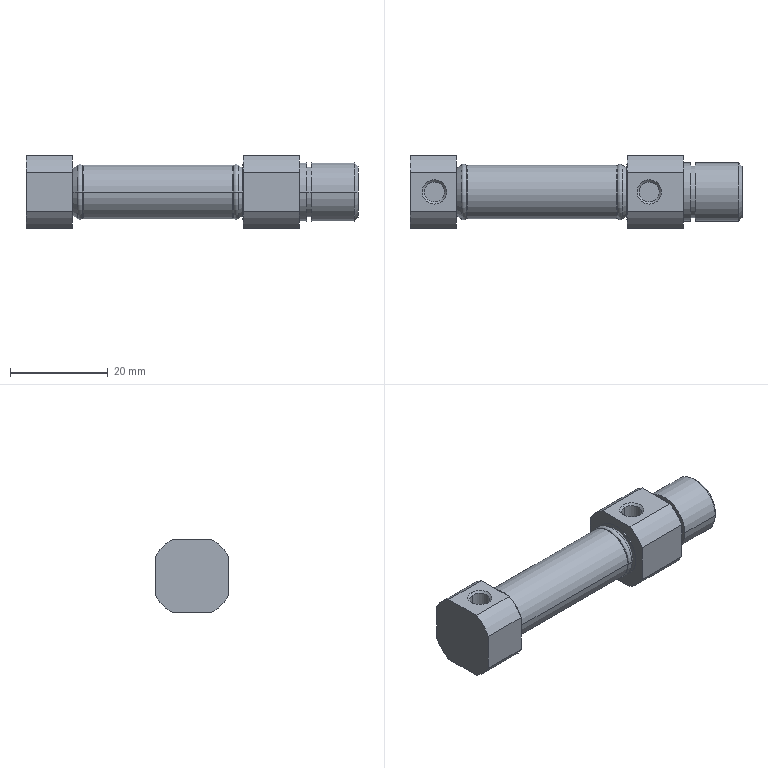Component | SolidWorks | MI10x10U(0)+()-1_MI 10x10-U_c-1 | 1 solid | 69 faces | box 68 x 15 x 15 mm | volume 6775 mm3 | cylinder 28 | plane 23 | cone 14 | torus 4 | commonest cylinder face diameters 17 x8 4.134 x4 11.4 x4 12 x4 9.6 x2 4 x2 11 x2 10.5 x2
build123d program:
from build123d import *

# Parameters (mm, degrees)
SKETCH3_W          = 30
SKETCH3_H          = 30
SKETCH3_W_2        = 15
SKETCH3_H_2        = 15
CUT_EXTRUDE1_DEPTH = 11.5
SKETCH4_W          = 30
SKETCH4_H          = 30
SKETCH4_W_2        = 15
SKETCH4_H_2        = 15
CUT_EXTRUDE2_DEPTH = 9.5
HOLE1_D            = 4.134
HOLE1_DEPTH        = 5
HOLE1_CSINK_D      = 5
HOLE1_CSINK_ANGLE  = 90
HOLE2_D            = 4.134
HOLE2_DEPTH        = 5
HOLE2_CSINK_D      = 5
HOLE2_CSINK_ANGLE  = 90


with BuildPart() as part:
    # Sketch1 → Revolve1 (revolve)
    with BuildSketch(Plane.XY, mode=Mode.PRIVATE) as revolve1_sk:
        Polygon((-12, 0), (-12, 5.233), (-11.233, 6), (-2.4, 6), (-2.4, 5.25), (-1.5, 5.25), (-1.5, 6), (0, 6), (0, 0), align=None)
    revolve(revolve1_sk.sketch.rotate(Axis((0, 0, 0), (-1, 0, 0)), 270), axis=Axis((0, 0, 0), (-1, 0, 0)))

    # Sketch2 → Revolve2 (revolve)
    with BuildSketch(Plane.XY, mode=Mode.PRIVATE) as revolve2_sk:
        with BuildLine():
            Line((0, 0), (0, 8.5))
            Line((0, 8.5), (11.5, 8.5))
            Line((11.5, 8.5), (11.5, 5.7))
            Line((11.5, 5.7), (11.6, 5.7))
            Line((11.6, 5.7), (11.6, 4.9))
            Line((11.6, 4.9), (12.5, 5.5))
            ThreePointArc((12.5, 5.5), (13, 5.7), (13.5, 5.5))
            Line((13.5, 5.5), (13.5, 5.3))
            Line((13.5, 5.3), (13.7, 5.5))
            Line((13.7, 5.5), (44.3, 5.5))
            Line((44.3, 5.5), (44.5, 5.3))
            Line((44.5, 5.3), (44.5, 5.5))
            ThreePointArc((44.5, 5.5), (45, 5.7), (45.5, 5.5))
            Line((45.5, 5.5), (46.4, 4.9))
            Line((46.4, 4.9), (46.4, 5.7))
            Line((46.4, 5.7), (46.5, 5.7))
            Line((46.5, 5.7), (46.5, 8.5))
            Line((46.5, 8.5), (56, 8.5))
            Line((56, 8.5), (56, 0))
            Line((56, 0), (0, 0))
        make_face()
    revolve(revolve2_sk.sketch.rotate(Axis((56, 0, 0), (-1, 0, 0)), 270), axis=Axis((56, 0, 0), (-1, 0, 0)))

    # Sketch3 → Cut-Extrude1 (cut)
    with BuildSketch(Plane(origin=(0, 0, 0), x_dir=(0, 0, -1), z_dir=(1, 0, 0))):
        Rectangle(SKETCH3_W, SKETCH3_H)
        Rectangle(SKETCH3_W_2, SKETCH3_H_2, mode=Mode.SUBTRACT)
    extrude(amount=CUT_EXTRUDE1_DEPTH, mode=Mode.SUBTRACT)

    # Sketch4 → Cut-Extrude2 (cut)
    with BuildSketch(Plane(origin=(56, 0, 0), x_dir=(0, 0, -1), z_dir=(1, 0, 0))):
        Rectangle(SKETCH4_W, SKETCH4_H)
        Rectangle(SKETCH4_W_2, SKETCH4_H_2, mode=Mode.SUBTRACT)
    extrude(amount=-CUT_EXTRUDE2_DEPTH, mode=Mode.SUBTRACT)

    # Hole1
    with Locations(Plane(origin=(0, 7.5, 0), x_dir=(1, 0, 0), z_dir=(0, 1, 0))):
        with Locations((7, 0)):
            CounterSinkHole(HOLE1_D / 2, HOLE1_CSINK_D / 2, depth=HOLE1_DEPTH, counter_sink_angle=HOLE1_CSINK_ANGLE)

    # Hole2
    with Locations(Plane(origin=(0, 7.5, 0), x_dir=(1, 0, 0), z_dir=(0, 1, 0))):
        with Locations((51, 0)):
            CounterSinkHole(HOLE2_D / 2, HOLE2_CSINK_D / 2, depth=HOLE2_DEPTH, counter_sink_angle=HOLE2_CSINK_ANGLE)

    # Sketch9 → Cut-Revolve1 (revolve, cut)
    with BuildSketch(Plane.XY, mode=Mode.PRIVATE) as cut_revolve1_sk:
        Polygon((-17, 0), (-17, 2), (18, 2), (18, 4.8), (41, 4.8), (41, 0), align=None)
    revolve(cut_revolve1_sk.sketch.rotate(Axis((41, 0, 0), (-1, 0, 0)), 270), axis=Axis((41, 0, 0), (-1, 0, 0)), mode=Mode.SUBTRACT)


solid = part.part

# Placed as in the assembly
solid = solid.moved(Location((-19.325, 30.452, 72.77), (-90, 0, 180)))